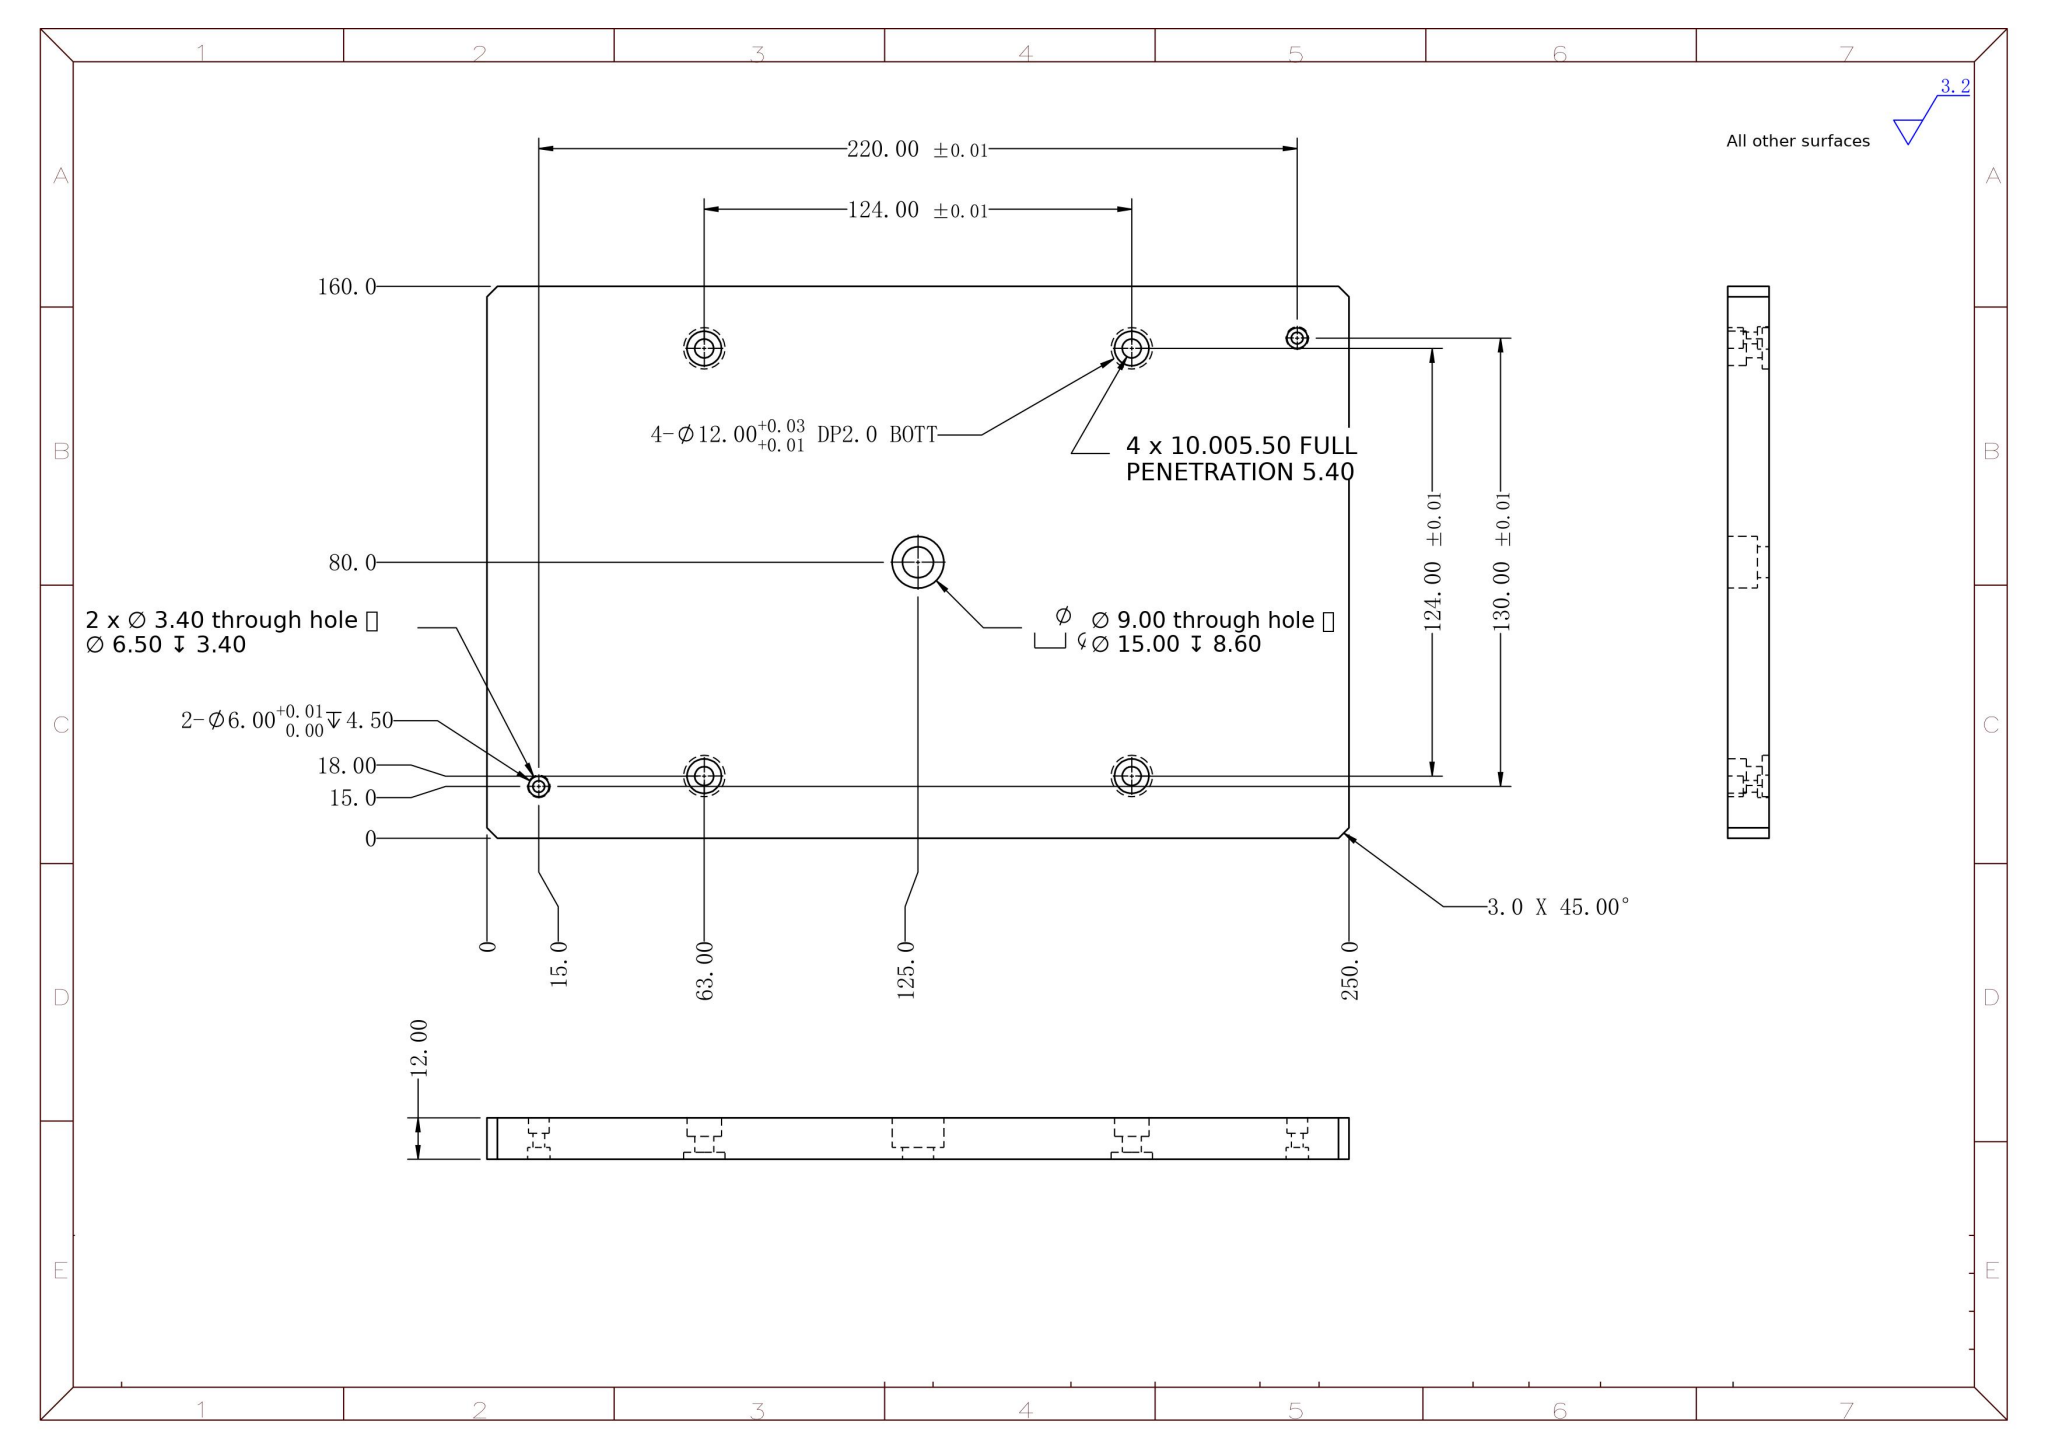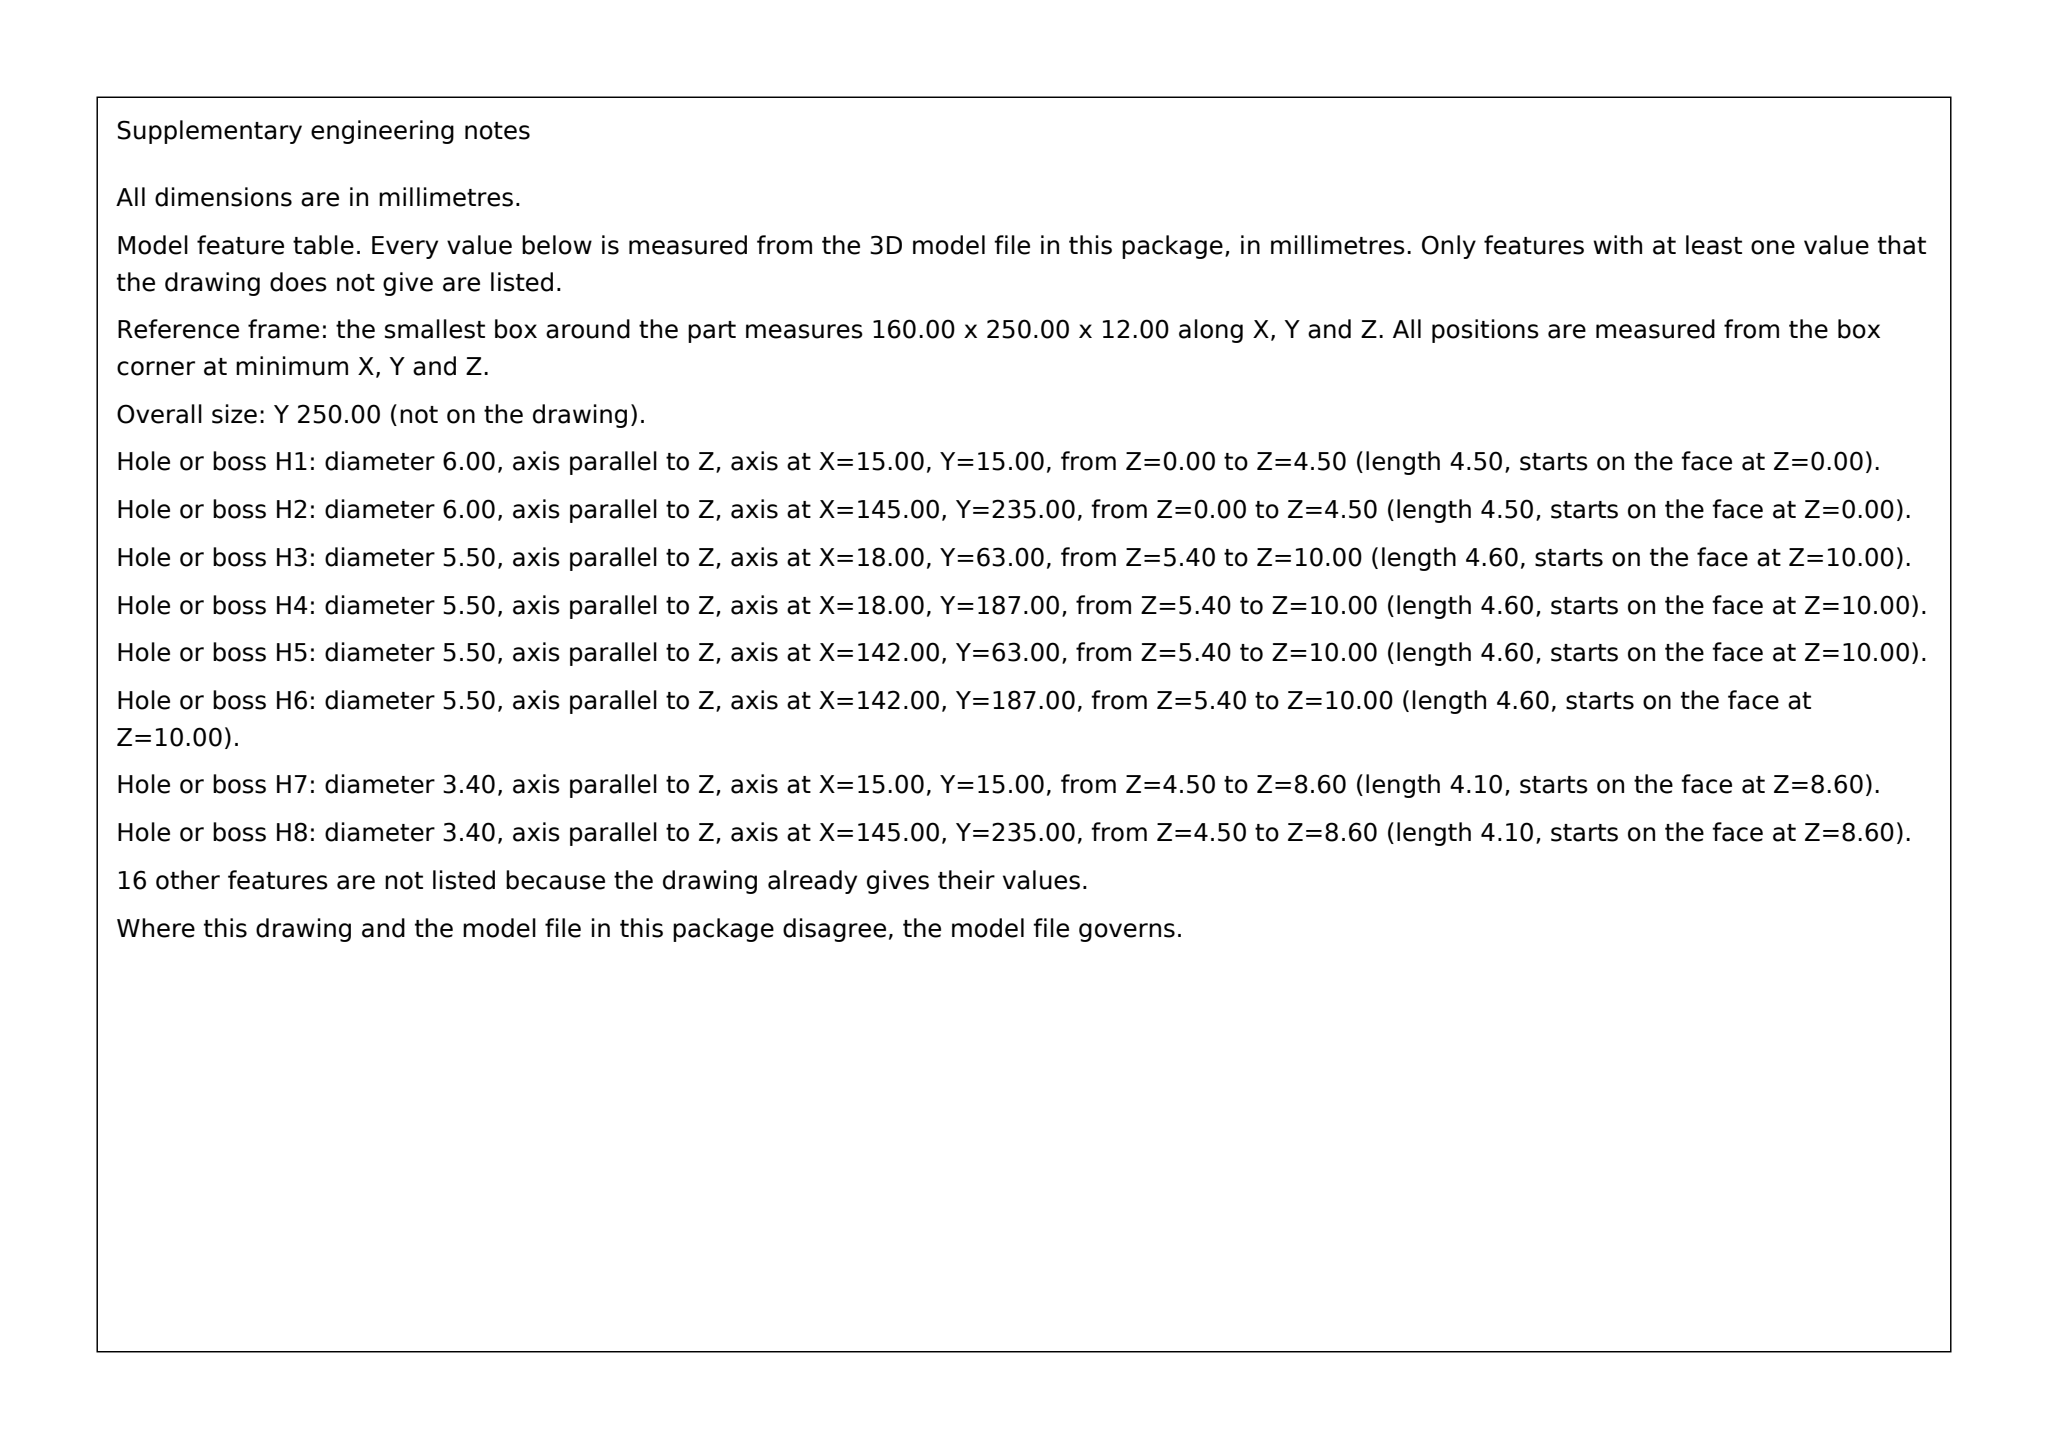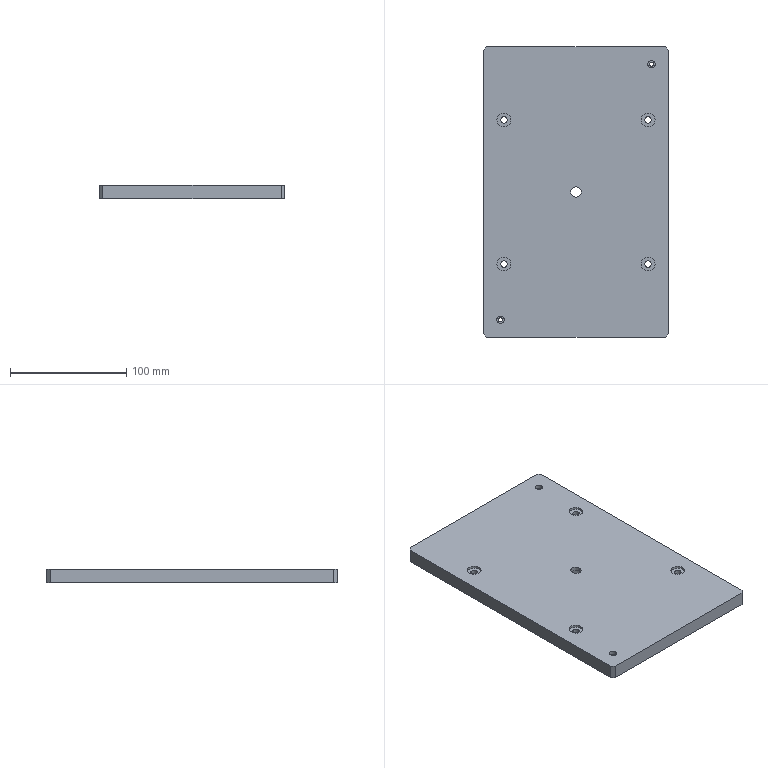Part | SolidWorks | mm | 1 solid | 63 faces | box 160 x 250 x 12 mm | volume 474455 mm3 | cylinder 40 | plane 23 | commonest cylinder face diameters 10.001 x8 5.5 x8 12 x8 6.5 x4 3.4 x4 6 x4 15 x2 9 x2
build123d program:
from build123d import *

# Parameters (mm, degrees)
SKETCH1_W                                       = 160
SKETCH1_H                                       = 250
BOSS_EXTRUDE1_DEPTH                             = 6
SKETCH2_R                                       = 6
CUT_EXTRUDE1_DEPTH                              = 2
M5_HEX_SOCKET_HEAD_CAP_SCREW_CBORE1_D           = 5.5
M5_HEX_SOCKET_HEAD_CAP_SCREW_CBORE1_CBORE_D     = 10.001
M5_HEX_SOCKET_HEAD_CAP_SCREW_CBORE1_CBORE_DEPTH = 5.4
CHAMFER1_SIZE                                   = 3
SKETCH16_R                                      = 3
CUT_EXTRUDE4_DEPTH                              = 4.5
M8_HEX_SOCKET_HEAD_CAP_SCREW_CBORE1_D           = 9
M8_HEX_SOCKET_HEAD_CAP_SCREW_CBORE1_CBORE_D     = 15
M8_HEX_SOCKET_HEAD_CAP_SCREW_CBORE1_CBORE_DEPTH = 8.6
M3_HEX_SOCKET_HEAD_CAP_SCREW_CBORE1_D           = 3.4
M3_HEX_SOCKET_HEAD_CAP_SCREW_CBORE1_CBORE_D     = 6.5
M3_HEX_SOCKET_HEAD_CAP_SCREW_CBORE1_CBORE_DEPTH = 3.4


with BuildPart() as part:
    # Sketch1 → Boss-Extrude1 (new, symmetric)
    with BuildSketch(Plane.XY):
        Rectangle(SKETCH1_W, SKETCH1_H)
    extrude(amount=BOSS_EXTRUDE1_DEPTH, both=True)

    # Sketch2 → Cut-Extrude1 (cut)
    with BuildSketch(Plane.XY.offset(6)):
        with Locations((-62, 62)):
            Circle(SKETCH2_R)
        with Locations((62, 62)):
            Circle(SKETCH2_R)
        with Locations((-62, -62)):
            Circle(SKETCH2_R)
        with Locations((62, -62)):
            Circle(SKETCH2_R)
    extrude(amount=-CUT_EXTRUDE1_DEPTH, mode=Mode.SUBTRACT)

    # M5 Hex Socket Head Cap Screw CBORE1 (through all)
    with Locations(Plane(origin=(0, 0, -6), x_dir=(-1, 0, 0), z_dir=(0, 0, -1))):
        with Locations((62, -62), (-62, -62), (62, 62), (-62, 62)):
            CounterBoreHole(M5_HEX_SOCKET_HEAD_CAP_SCREW_CBORE1_D / 2, M5_HEX_SOCKET_HEAD_CAP_SCREW_CBORE1_CBORE_D / 2, M5_HEX_SOCKET_HEAD_CAP_SCREW_CBORE1_CBORE_DEPTH)

    # Chamfer1
    chamfer1_edges = [part.edges().sort_by_distance(p)[0] for p in [
        (80, -125, 0),
        (-80, -125, 0),
        (-80, 125, 0),
        (80, 125, 0),
    ]]
    chamfer(chamfer1_edges, length=CHAMFER1_SIZE)

    # Sketch16 → Cut-Extrude4 (cut)
    with BuildSketch(Plane(origin=(0, 0, -6), x_dir=(-1, 0, 0), z_dir=(0, 0, -1))):
        with Locations((-65, 110)):
            Circle(SKETCH16_R)
        with Locations((65, -110)):
            Circle(SKETCH16_R)
    extrude(amount=-CUT_EXTRUDE4_DEPTH, mode=Mode.SUBTRACT)

    # M8 Hex Socket Head Cap Screw CBORE1 (through all)
    with Locations(Plane(origin=(0, 0, -6), x_dir=(-1, 0, 0), z_dir=(0, 0, -1))):
        with Locations((0, 0)):
            CounterBoreHole(M8_HEX_SOCKET_HEAD_CAP_SCREW_CBORE1_D / 2, M8_HEX_SOCKET_HEAD_CAP_SCREW_CBORE1_CBORE_D / 2, M8_HEX_SOCKET_HEAD_CAP_SCREW_CBORE1_CBORE_DEPTH)

    # M3 Hex Socket Head Cap Screw CBORE1 (through all)
    with Locations(Plane.XY.offset(6)):
        with Locations((65, 110), (-65, -110)):
            CounterBoreHole(M3_HEX_SOCKET_HEAD_CAP_SCREW_CBORE1_D / 2, M3_HEX_SOCKET_HEAD_CAP_SCREW_CBORE1_CBORE_D / 2, M3_HEX_SOCKET_HEAD_CAP_SCREW_CBORE1_CBORE_DEPTH)


solid = part.part